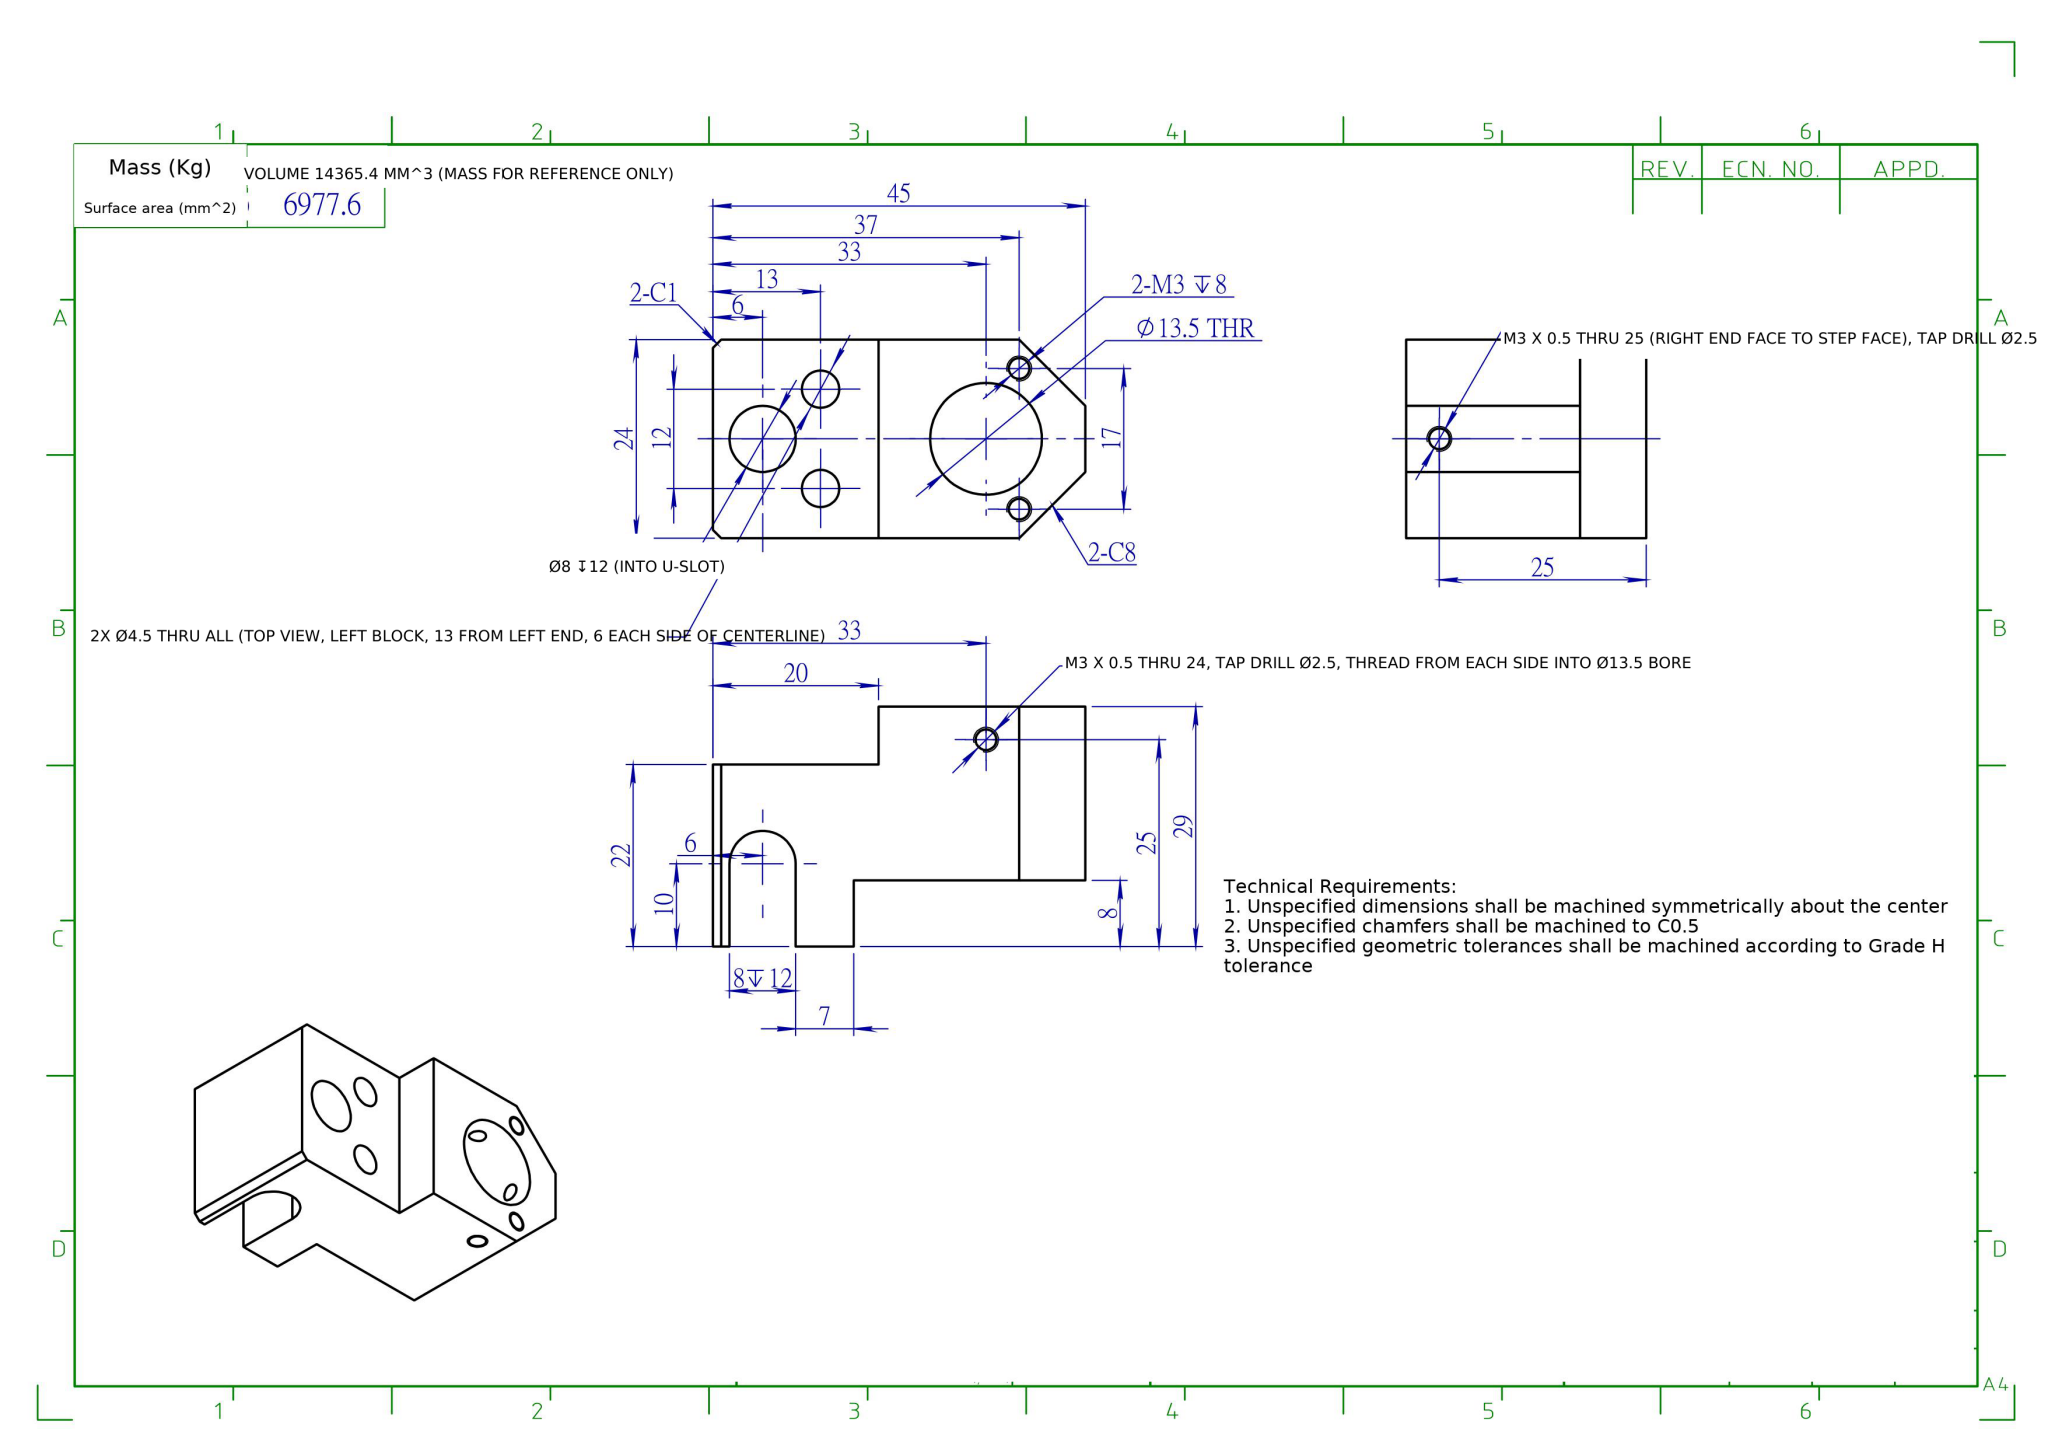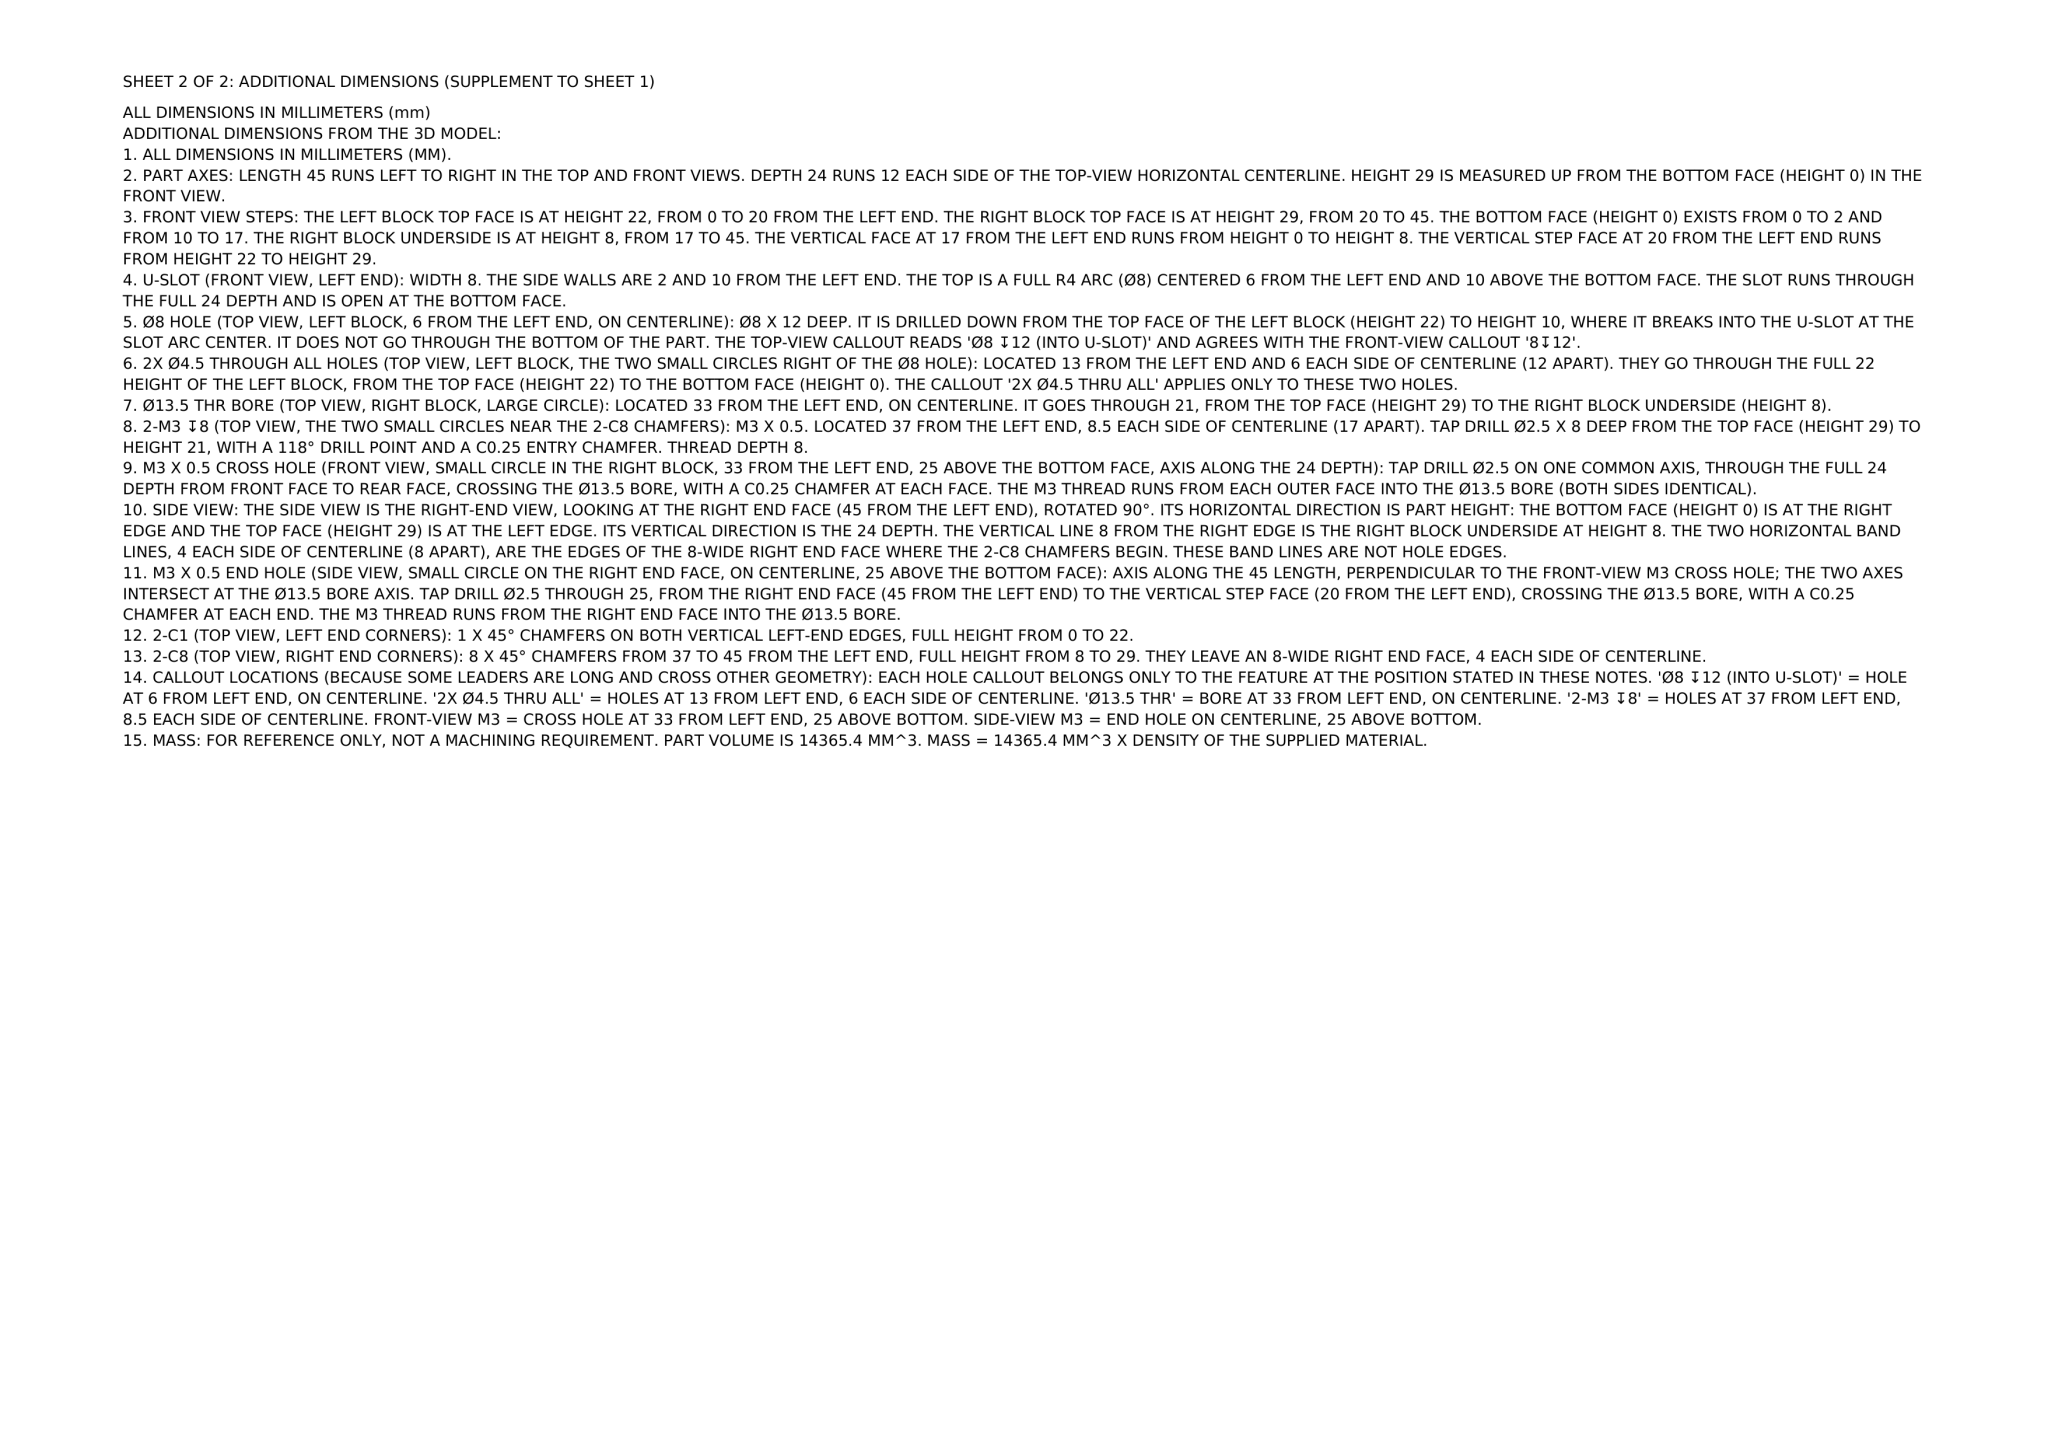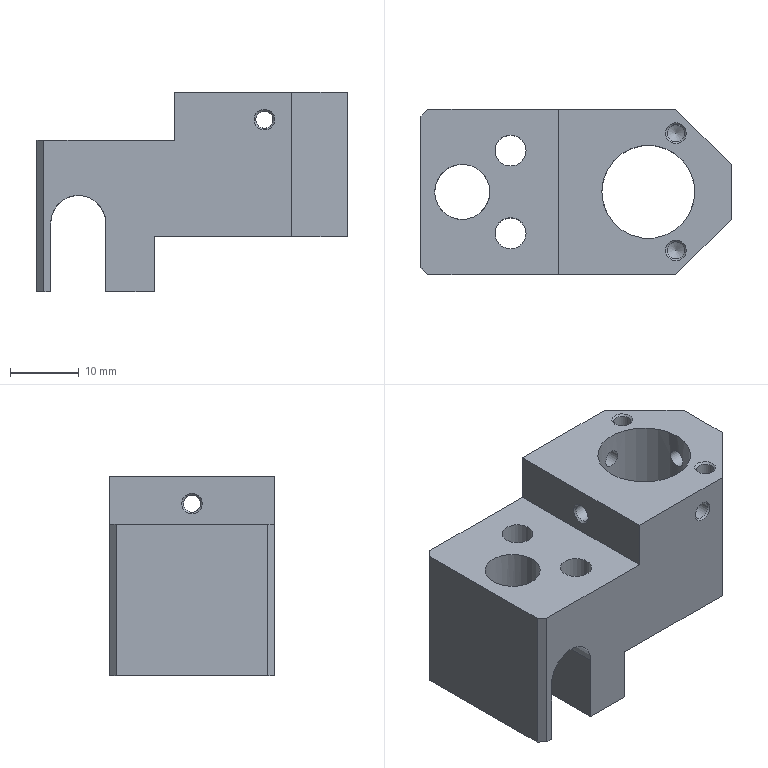Part | NX | mm | 1 solid | 37 faces | box 45 x 24 x 29 mm | volume 14365 mm3 | plane 17 | cylinder 12 | cone 8 | commonest cylinder face diameters 2.5 x6 8 x3 4.5 x2 13.5 x1